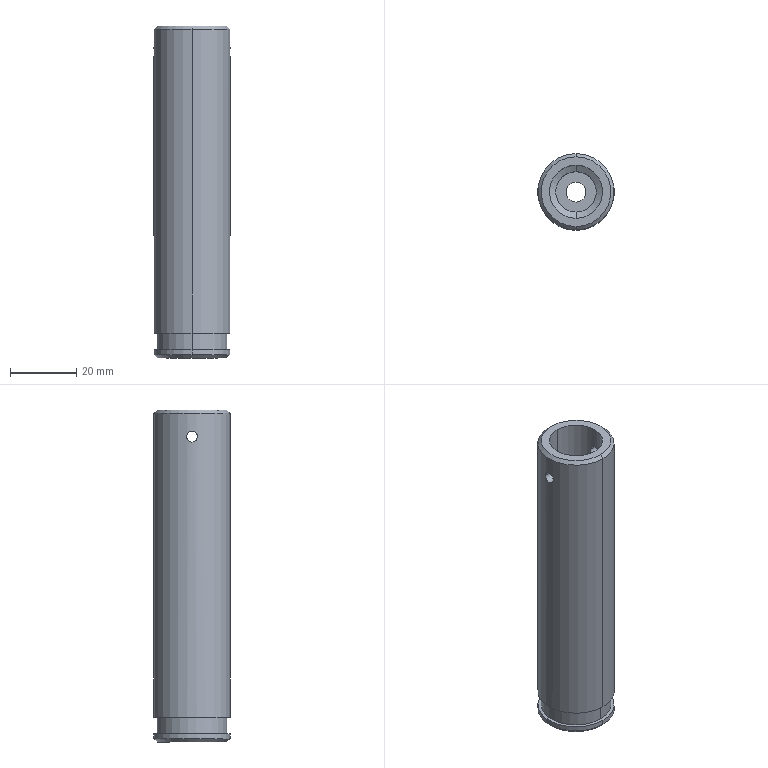Component | SolidWorks | DZ.KX.203-TC1505-20-18-05-98-1 | 1 solid | 30 faces | box 23 x 23 x 100 mm | volume 30575 mm3 | cylinder 18 | cone 6 | plane 6 | commonest cylinder face diameters 3.3 x4 23 x4 10.5 x2 21 x2 16 x2 12.2 x2 6 x2 | material Cast Stainless Steel
STEP:
#1=COLOUR_RGB('',0.7922,0.8196,0.9333);
#2=FILL_AREA_STYLE_COLOUR('',#1);
#3=FILL_AREA_STYLE('',(#2));
#4=SURFACE_STYLE_FILL_AREA(#3);
#5=SURFACE_SIDE_STYLE('',(#4));
#6=SURFACE_STYLE_USAGE(.BOTH.,#5);
#7=PRESENTATION_STYLE_ASSIGNMENT((#6));
#8=CARTESIAN_POINT('',(11.634,-31.784,4.53));
#9=VERTEX_POINT('',#8);
#10=CARTESIAN_POINT('',(11.634,-32.611,4.53));
#11=VERTEX_POINT('',#10);
#12=CARTESIAN_POINT('',(11.634,-32.197,4.53));
#13=DIRECTION('',(-0.,0.,1.));
#14=DIRECTION('',(0.,-1.,0.));
#15=AXIS2_PLACEMENT_3D('',#12,#13,#14);
#16=CIRCLE('',#15,0.4134);
#17=EDGE_CURVE('',#9,#11,#16,.T.);
#18=ORIENTED_EDGE('',*,*,#17,.F.);
#19=CARTESIAN_POINT('',(11.634,-31.744,4.491));
#20=VERTEX_POINT('',#19);
#21=CARTESIAN_POINT('',(11.634,-31.744,4.491));
#22=DIRECTION('',(-0.,0.7071,-0.7071));
#23=VECTOR('',#22,39.37);
#24=LINE('',#21,#23);
#25=EDGE_CURVE('',#9,#20,#24,.T.);
#26=ORIENTED_EDGE('',*,*,#25,.T.);
#27=CARTESIAN_POINT('',(11.634,-32.65,4.491));
#28=VERTEX_POINT('',#27);
#29=CARTESIAN_POINT('',(11.634,-32.197,4.491));
#30=DIRECTION('',(0.,-0.,-1.));
#31=DIRECTION('',(0.,-1.,0.));
#32=AXIS2_PLACEMENT_3D('',#29,#30,#31);
#33=CIRCLE('',#32,0.4528);
#34=EDGE_CURVE('',#28,#20,#33,.T.);
#35=ORIENTED_EDGE('',*,*,#34,.F.);
#36=CARTESIAN_POINT('',(11.634,-32.65,4.491));
#37=DIRECTION('',(0.,-0.7071,-0.7071));
#38=VECTOR('',#37,39.37);
#39=LINE('',#36,#38);
#40=EDGE_CURVE('',#11,#28,#39,.T.);
#41=ORIENTED_EDGE('',*,*,#40,.F.);
#42=EDGE_LOOP('',(#18,#26,#35,#41));
#43=FACE_OUTER_BOUND('',#42,.T.);
#44=CARTESIAN_POINT('',(11.634,-32.197,4.491));
#45=DIRECTION('',(0.,-0.,-1.));
#46=DIRECTION('',(0.,-1.,0.));
#47=AXIS2_PLACEMENT_3D('',#44,#45,#46);
#48=CONICAL_SURFACE('',#47,0.4528,0.7854);
#49=ADVANCED_FACE('',(#43),#48,.T.);
#50=CARTESIAN_POINT('',(11.634,-32.611,0.5929));
#51=VERTEX_POINT('',#50);
#52=CARTESIAN_POINT('',(11.634,-31.784,0.5929));
#53=VERTEX_POINT('',#52);
#54=CARTESIAN_POINT('',(11.634,-32.197,0.5929));
#55=DIRECTION('',(0.,-0.,-1.));
#56=DIRECTION('',(0.,-1.,0.));
#57=AXIS2_PLACEMENT_3D('',#54,#55,#56);
#58=CIRCLE('',#57,0.4134);
#59=EDGE_CURVE('',#51,#53,#58,.T.);
#60=ORIENTED_EDGE('',*,*,#59,.F.);
#61=CARTESIAN_POINT('',(11.634,-32.65,0.6323));
#62=VERTEX_POINT('',#61);
#63=CARTESIAN_POINT('',(11.634,-32.611,0.5929));
#64=DIRECTION('',(0.,-0.7071,0.7071));
#65=VECTOR('',#64,39.37);
#66=LINE('',#63,#65);
#67=EDGE_CURVE('',#51,#62,#66,.T.);
#68=ORIENTED_EDGE('',*,*,#67,.T.);
#69=CARTESIAN_POINT('',(11.634,-31.744,0.6323));
#70=VERTEX_POINT('',#69);
#71=CARTESIAN_POINT('',(11.634,-32.197,0.6323));
#72=DIRECTION('',(-0.,0.,1.));
#73=DIRECTION('',(0.,-1.,0.));
#74=AXIS2_PLACEMENT_3D('',#71,#72,#73);
#75=CIRCLE('',#74,0.4528);
#76=EDGE_CURVE('',#70,#62,#75,.T.);
#77=ORIENTED_EDGE('',*,*,#76,.F.);
#78=CARTESIAN_POINT('',(11.634,-31.784,0.5929));
#79=DIRECTION('',(-0.,0.7071,0.7071));
#80=VECTOR('',#79,39.37);
#81=LINE('',#78,#80);
#82=EDGE_CURVE('',#53,#70,#81,.T.);
#83=ORIENTED_EDGE('',*,*,#82,.F.);
#84=EDGE_LOOP('',(#60,#68,#77,#83));
#85=FACE_OUTER_BOUND('',#84,.T.);
#86=CARTESIAN_POINT('',(11.634,-32.197,0.5929));
#87=DIRECTION('',(-0.,0.,1.));
#88=DIRECTION('',(0.,1.,-0.));
#89=AXIS2_PLACEMENT_3D('',#86,#87,#88);
#90=CONICAL_SURFACE('',#89,0.4134,0.7854);
#91=ADVANCED_FACE('',(#85),#90,.T.);
#92=CARTESIAN_POINT('',(11.634,-31.99,1.183));
#93=VERTEX_POINT('',#92);
#94=CARTESIAN_POINT('',(11.634,-32.404,1.183));
#95=VERTEX_POINT('',#94);
#96=CARTESIAN_POINT('',(11.634,-32.197,1.183));
#97=DIRECTION('',(0.,-0.,-1.));
#98=DIRECTION('',(0.,-1.,0.));
#99=AXIS2_PLACEMENT_3D('',#96,#97,#98);
#100=CIRCLE('',#99,0.2067);
#101=EDGE_CURVE('',#93,#95,#100,.T.);
#102=ORIENTED_EDGE('',*,*,#101,.F.);
#103=CARTESIAN_POINT('',(11.634,-31.99,0.5929));
#104=VERTEX_POINT('',#103);
#105=CARTESIAN_POINT('',(11.634,-31.99,0.5929));
#106=DIRECTION('',(0.,-0.,-1.));
#107=VECTOR('',#106,39.37);
#108=LINE('',#105,#107);
#109=EDGE_CURVE('',#93,#104,#108,.T.);
#110=ORIENTED_EDGE('',*,*,#109,.T.);
#111=CARTESIAN_POINT('',(11.634,-32.404,0.5929));
#112=VERTEX_POINT('',#111);
#113=CARTESIAN_POINT('',(11.634,-32.197,0.5929));
#114=DIRECTION('',(0.,-0.,-1.));
#115=DIRECTION('',(0.,-1.,0.));
#116=AXIS2_PLACEMENT_3D('',#113,#114,#115);
#117=CIRCLE('',#116,0.2067);
#118=EDGE_CURVE('',#104,#112,#117,.T.);
#119=ORIENTED_EDGE('',*,*,#118,.T.);
#120=CARTESIAN_POINT('',(11.634,-32.404,0.5929));
#121=DIRECTION('',(0.,-0.,-1.));
#122=VECTOR('',#121,39.37);
#123=LINE('',#120,#122);
#124=EDGE_CURVE('',#95,#112,#123,.T.);
#125=ORIENTED_EDGE('',*,*,#124,.F.);
#126=EDGE_LOOP('',(#102,#110,#119,#125));
#127=FACE_OUTER_BOUND('',#126,.T.);
#128=CARTESIAN_POINT('',(11.634,-32.197,0.5929));
#129=DIRECTION('',(0.,-0.,-1.));
#130=DIRECTION('',(0.,-1.,0.));
#131=AXIS2_PLACEMENT_3D('',#128,#129,#130);
#132=CYLINDRICAL_SURFACE('',#131,0.2067);
#133=ADVANCED_FACE('',(#127),#132,.F.);
#134=CARTESIAN_POINT('',(11.634,-32.611,0.8882));
#135=VERTEX_POINT('',#134);
#136=CARTESIAN_POINT('',(11.634,-31.784,0.8882));
#137=VERTEX_POINT('',#136);
#138=CARTESIAN_POINT('',(11.634,-32.197,0.8882));
#139=DIRECTION('',(0.,-0.,-1.));
#140=DIRECTION('',(0.,-1.,0.));
#141=AXIS2_PLACEMENT_3D('',#138,#139,#140);
#142=CIRCLE('',#141,0.4134);
#143=EDGE_CURVE('',#135,#137,#142,.T.);
#144=ORIENTED_EDGE('',*,*,#143,.T.);
#145=CARTESIAN_POINT('',(11.634,-31.784,0.6913));
#146=VERTEX_POINT('',#145);
#147=CARTESIAN_POINT('',(11.634,-31.784,0.8882));
#148=DIRECTION('',(0.,-0.,-1.));
#149=VECTOR('',#148,39.37);
#150=LINE('',#147,#149);
#151=EDGE_CURVE('',#137,#146,#150,.T.);
#152=ORIENTED_EDGE('',*,*,#151,.T.);
#153=CARTESIAN_POINT('',(11.634,-32.611,0.6913));
#154=VERTEX_POINT('',#153);
#155=CARTESIAN_POINT('',(11.634,-32.197,0.6913));
#156=DIRECTION('',(0.,-0.,-1.));
#157=DIRECTION('',(0.,-1.,0.));
#158=AXIS2_PLACEMENT_3D('',#155,#156,#157);
#159=CIRCLE('',#158,0.4134);
#160=EDGE_CURVE('',#154,#146,#159,.T.);
#161=ORIENTED_EDGE('',*,*,#160,.F.);
#162=CARTESIAN_POINT('',(11.634,-32.611,0.8882));
#163=DIRECTION('',(0.,-0.,-1.));
#164=VECTOR('',#163,39.37);
#165=LINE('',#162,#164);
#166=EDGE_CURVE('',#135,#154,#165,.T.);
#167=ORIENTED_EDGE('',*,*,#166,.F.);
#168=EDGE_LOOP('',(#144,#152,#161,#167));
#169=FACE_OUTER_BOUND('',#168,.T.);
#170=CARTESIAN_POINT('',(11.634,-32.197,0.8882));
#171=DIRECTION('',(0.,-0.,-1.));
#172=DIRECTION('',(0.,-1.,0.));
#173=AXIS2_PLACEMENT_3D('',#170,#171,#172);
#174=CYLINDRICAL_SURFACE('',#173,0.4134);
#175=ADVANCED_FACE('',(#169),#174,.T.);
#176=CARTESIAN_POINT('',(12.082,-32.262,4.215));
#177=VERTEX_POINT('',#176);
#178=CARTESIAN_POINT('',(12.082,-32.132,4.215));
#179=VERTEX_POINT('',#178);
#180=CARTESIAN_POINT('',(12.082,-32.262,4.215));
#181=CARTESIAN_POINT('',(12.082,-32.262,4.219));
#182=CARTESIAN_POINT('',(12.082,-32.262,4.223));
#183=CARTESIAN_POINT('',(12.082,-32.26,4.232));
#184=CARTESIAN_POINT('',(12.082,-32.259,4.236));
#185=CARTESIAN_POINT('',(12.083,-32.255,4.244));
#186=CARTESIAN_POINT('',(12.083,-32.254,4.247));
#187=CARTESIAN_POINT('',(12.084,-32.249,4.255));
#188=CARTESIAN_POINT('',(12.084,-32.246,4.258));
#189=CARTESIAN_POINT('',(12.085,-32.237,4.267));
#190=CARTESIAN_POINT('',(12.085,-32.23,4.272));
#191=CARTESIAN_POINT('',(12.086,-32.214,4.278));
#192=CARTESIAN_POINT('',(12.087,-32.206,4.28));
#193=CARTESIAN_POINT('',(12.087,-32.193,4.28));
#194=CARTESIAN_POINT('',(12.087,-32.189,4.279));
#195=CARTESIAN_POINT('',(12.086,-32.18,4.278));
#196=CARTESIAN_POINT('',(12.086,-32.176,4.277));
#197=CARTESIAN_POINT('',(12.086,-32.168,4.273));
#198=CARTESIAN_POINT('',(12.085,-32.165,4.271));
#199=CARTESIAN_POINT('',(12.085,-32.157,4.267));
#200=CARTESIAN_POINT('',(12.085,-32.154,4.264));
#201=CARTESIAN_POINT('',(12.084,-32.145,4.255));
#202=CARTESIAN_POINT('',(12.083,-32.14,4.248));
#203=CARTESIAN_POINT('',(12.082,-32.134,4.232));
#204=CARTESIAN_POINT('',(12.082,-32.132,4.223));
#205=CARTESIAN_POINT('',(12.082,-32.132,4.215));
#206=B_SPLINE_CURVE_WITH_KNOTS('',3,(#180,#181,#182,#183,#184,#185,#186,#187,#188,#189,#190,#191,#192,#193,#194,#195,#196,#197,#198,#199,#200,#201,#202,#203,#204,#205),.UNSPECIFIED.,.F.,.F.,(4,2,2,2,2,2,2,2,2,2,2,2,4),(0.007748,0.008071,0.008394,0.008717,0.009039,0.009685,0.01033,0.01065,0.01098,0.0113,0.01162,0.01227,0.01291),.UNSPECIFIED.);
#207=EDGE_CURVE('',#177,#179,#206,.T.);
#208=ORIENTED_EDGE('',*,*,#207,.F.);
#209=CARTESIAN_POINT('',(11.942,-32.262,4.215));
#210=VERTEX_POINT('',#209);
#211=CARTESIAN_POINT('',(11.142,-32.262,4.215));
#212=DIRECTION('',(-1.,-0.,-0.));
#213=VECTOR('',#212,39.37);
#214=LINE('',#211,#213);
#215=EDGE_CURVE('',#177,#210,#214,.T.);
#216=ORIENTED_EDGE('',*,*,#215,.T.);
#217=CARTESIAN_POINT('',(11.942,-32.132,4.215));
#218=VERTEX_POINT('',#217);
#219=CARTESIAN_POINT('',(11.942,-32.132,4.215));
#220=CARTESIAN_POINT('',(11.942,-32.132,4.219));
#221=CARTESIAN_POINT('',(11.942,-32.133,4.223));
#222=CARTESIAN_POINT('',(11.942,-32.134,4.232));
#223=CARTESIAN_POINT('',(11.943,-32.135,4.236));
#224=CARTESIAN_POINT('',(11.943,-32.139,4.244));
#225=CARTESIAN_POINT('',(11.944,-32.141,4.248));
#226=CARTESIAN_POINT('',(11.945,-32.145,4.255));
#227=CARTESIAN_POINT('',(11.945,-32.148,4.258));
#228=CARTESIAN_POINT('',(11.946,-32.157,4.267));
#229=CARTESIAN_POINT('',(11.947,-32.164,4.272));
#230=CARTESIAN_POINT('',(11.948,-32.18,4.278));
#231=CARTESIAN_POINT('',(11.949,-32.189,4.28));
#232=CARTESIAN_POINT('',(11.949,-32.201,4.28));
#233=CARTESIAN_POINT('',(11.949,-32.206,4.279));
#234=CARTESIAN_POINT('',(11.948,-32.214,4.278));
#235=CARTESIAN_POINT('',(11.948,-32.218,4.277));
#236=CARTESIAN_POINT('',(11.947,-32.23,4.272));
#237=CARTESIAN_POINT('',(11.946,-32.237,4.267));
#238=CARTESIAN_POINT('',(11.945,-32.246,4.258));
#239=CARTESIAN_POINT('',(11.945,-32.249,4.255));
#240=CARTESIAN_POINT('',(11.944,-32.253,4.248));
#241=CARTESIAN_POINT('',(11.943,-32.255,4.244));
#242=CARTESIAN_POINT('',(11.943,-32.259,4.236));
#243=CARTESIAN_POINT('',(11.942,-32.26,4.232));
#244=CARTESIAN_POINT('',(11.942,-32.262,4.224));
#245=CARTESIAN_POINT('',(11.942,-32.262,4.219));
#246=CARTESIAN_POINT('',(11.942,-32.262,4.215));
#247=B_SPLINE_CURVE_WITH_KNOTS('',3,(#219,#220,#221,#222,#223,#224,#225,#226,#227,#228,#229,#230,#231,#232,#233,#234,#235,#236,#237,#238,#239,#240,#241,#242,#243,#244,#245,#246),.UNSPECIFIED.,.F.,.F.,(4,2,2,2,2,2,2,2,2,2,2,2,2,4),(0.,0.0003233,0.0006466,0.0009699,0.001293,0.00194,0.002586,0.00291,0.003233,0.003879,0.004203,0.004526,0.004849,0.005173),.UNSPECIFIED.);
#248=EDGE_CURVE('',#218,#210,#247,.T.);
#249=ORIENTED_EDGE('',*,*,#248,.F.);
#250=CARTESIAN_POINT('',(11.142,-32.132,4.215));
#251=DIRECTION('',(-1.,-0.,-0.));
#252=VECTOR('',#251,39.37);
#253=LINE('',#250,#252);
#254=EDGE_CURVE('',#179,#218,#253,.T.);
#255=ORIENTED_EDGE('',*,*,#254,.F.);
#256=EDGE_LOOP('',(#208,#216,#249,#255));
#257=FACE_OUTER_BOUND('',#256,.T.);
#258=CARTESIAN_POINT('',(11.142,-32.197,4.215));
#259=DIRECTION('',(-1.,-0.,-0.));
#260=DIRECTION('',(0.,1.,0.));
#261=AXIS2_PLACEMENT_3D('',#258,#259,#260);
#262=CYLINDRICAL_SURFACE('',#261,0.06496);
#263=ADVANCED_FACE('',(#257),#262,.F.);
#264=CARTESIAN_POINT('',(11.326,-32.262,4.215));
#265=VERTEX_POINT('',#264);
#266=CARTESIAN_POINT('',(11.326,-32.132,4.215));
#267=VERTEX_POINT('',#266);
#268=CARTESIAN_POINT('',(11.326,-32.262,4.215));
#269=CARTESIAN_POINT('',(11.326,-32.262,4.223));
#270=CARTESIAN_POINT('',(11.325,-32.26,4.232));
#271=CARTESIAN_POINT('',(11.324,-32.256,4.244));
#272=CARTESIAN_POINT('',(11.324,-32.253,4.248));
#273=CARTESIAN_POINT('',(11.323,-32.249,4.255));
#274=CARTESIAN_POINT('',(11.323,-32.246,4.258));
#275=CARTESIAN_POINT('',(11.322,-32.24,4.264));
#276=CARTESIAN_POINT('',(11.321,-32.237,4.267));
#277=CARTESIAN_POINT('',(11.321,-32.23,4.271));
#278=CARTESIAN_POINT('',(11.32,-32.226,4.273));
#279=CARTESIAN_POINT('',(11.319,-32.214,4.278));
#280=CARTESIAN_POINT('',(11.319,-32.206,4.28));
#281=CARTESIAN_POINT('',(11.319,-32.193,4.28));
#282=CARTESIAN_POINT('',(11.319,-32.189,4.279));
#283=CARTESIAN_POINT('',(11.319,-32.18,4.278));
#284=CARTESIAN_POINT('',(11.32,-32.176,4.277));
#285=CARTESIAN_POINT('',(11.32,-32.168,4.273));
#286=CARTESIAN_POINT('',(11.321,-32.165,4.271));
#287=CARTESIAN_POINT('',(11.321,-32.158,4.267));
#288=CARTESIAN_POINT('',(11.322,-32.154,4.264));
#289=CARTESIAN_POINT('',(11.323,-32.145,4.255));
#290=CARTESIAN_POINT('',(11.324,-32.14,4.248));
#291=CARTESIAN_POINT('',(11.325,-32.136,4.236));
#292=CARTESIAN_POINT('',(11.325,-32.134,4.232));
#293=CARTESIAN_POINT('',(11.326,-32.133,4.223));
#294=CARTESIAN_POINT('',(11.326,-32.132,4.219));
#295=CARTESIAN_POINT('',(11.326,-32.132,4.215));
#296=B_SPLINE_CURVE_WITH_KNOTS('',3,(#268,#269,#270,#271,#272,#273,#274,#275,#276,#277,#278,#279,#280,#281,#282,#283,#284,#285,#286,#287,#288,#289,#290,#291,#292,#293,#294,#295),.UNSPECIFIED.,.F.,.F.,(4,2,2,2,2,2,2,2,2,2,2,2,2,4),(0.005173,0.005819,0.006142,0.006465,0.006789,0.007112,0.007758,0.008081,0.008405,0.008728,0.009051,0.009697,0.01002,0.01034),.UNSPECIFIED.);
#297=EDGE_CURVE('',#265,#267,#296,.T.);
#298=ORIENTED_EDGE('',*,*,#297,.F.);
#299=CARTESIAN_POINT('',(11.186,-32.262,4.215));
#300=VERTEX_POINT('',#299);
#301=CARTESIAN_POINT('',(11.142,-32.262,4.215));
#302=DIRECTION('',(-1.,-0.,-0.));
#303=VECTOR('',#302,39.37);
#304=LINE('',#301,#303);
#305=EDGE_CURVE('',#265,#300,#304,.T.);
#306=ORIENTED_EDGE('',*,*,#305,.T.);
#307=CARTESIAN_POINT('',(11.186,-32.132,4.215));
#308=VERTEX_POINT('',#307);
#309=CARTESIAN_POINT('',(11.186,-32.132,4.215));
#310=CARTESIAN_POINT('',(11.186,-32.132,4.219));
#311=CARTESIAN_POINT('',(11.186,-32.133,4.223));
#312=CARTESIAN_POINT('',(11.185,-32.134,4.232));
#313=CARTESIAN_POINT('',(11.185,-32.135,4.236));
#314=CARTESIAN_POINT('',(11.185,-32.139,4.244));
#315=CARTESIAN_POINT('',(11.185,-32.141,4.247));
#316=CARTESIAN_POINT('',(11.184,-32.145,4.255));
#317=CARTESIAN_POINT('',(11.184,-32.148,4.258));
#318=CARTESIAN_POINT('',(11.183,-32.157,4.267));
#319=CARTESIAN_POINT('',(11.182,-32.164,4.272));
#320=CARTESIAN_POINT('',(11.181,-32.18,4.278));
#321=CARTESIAN_POINT('',(11.181,-32.189,4.28));
#322=CARTESIAN_POINT('',(11.181,-32.201,4.28));
#323=CARTESIAN_POINT('',(11.181,-32.206,4.279));
#324=CARTESIAN_POINT('',(11.181,-32.214,4.278));
#325=CARTESIAN_POINT('',(11.182,-32.218,4.277));
#326=CARTESIAN_POINT('',(11.182,-32.226,4.273));
#327=CARTESIAN_POINT('',(11.182,-32.23,4.271));
#328=CARTESIAN_POINT('',(11.183,-32.237,4.267));
#329=CARTESIAN_POINT('',(11.183,-32.24,4.264));
#330=CARTESIAN_POINT('',(11.184,-32.246,4.258));
#331=CARTESIAN_POINT('',(11.184,-32.249,4.255));
#332=CARTESIAN_POINT('',(11.185,-32.253,4.248));
#333=CARTESIAN_POINT('',(11.185,-32.256,4.244));
#334=CARTESIAN_POINT('',(11.185,-32.259,4.236));
#335=CARTESIAN_POINT('',(11.185,-32.26,4.232));
#336=CARTESIAN_POINT('',(11.186,-32.262,4.223));
#337=CARTESIAN_POINT('',(11.186,-32.262,4.219));
#338=CARTESIAN_POINT('',(11.186,-32.262,4.215));
#339=B_SPLINE_CURVE_WITH_KNOTS('',3,(#309,#310,#311,#312,#313,#314,#315,#316,#317,#318,#319,#320,#321,#322,#323,#324,#325,#326,#327,#328,#329,#330,#331,#332,#333,#334,#335,#336,#337,#338),.UNSPECIFIED.,.F.,.F.,(4,2,2,2,2,2,2,2,2,2,2,2,2,2,4),(0.,0.0003228,0.0006457,0.0009685,0.001291,0.001937,0.002583,0.002905,0.003228,0.003551,0.003874,0.004197,0.00452,0.004842,0.005165),.UNSPECIFIED.);
#340=EDGE_CURVE('',#308,#300,#339,.T.);
#341=ORIENTED_EDGE('',*,*,#340,.F.);
#342=CARTESIAN_POINT('',(11.142,-32.132,4.215));
#343=DIRECTION('',(-1.,-0.,-0.));
#344=VECTOR('',#343,39.37);
#345=LINE('',#342,#344);
#346=EDGE_CURVE('',#267,#308,#345,.T.);
#347=ORIENTED_EDGE('',*,*,#346,.F.);
#348=EDGE_LOOP('',(#298,#306,#341,#347));
#349=FACE_OUTER_BOUND('',#348,.T.);
#350=CARTESIAN_POINT('',(11.142,-32.197,4.215));
#351=DIRECTION('',(-1.,-0.,-0.));
#352=DIRECTION('',(0.,1.,0.));
#353=AXIS2_PLACEMENT_3D('',#350,#351,#352);
#354=CYLINDRICAL_SURFACE('',#353,0.06496);
#355=ADVANCED_FACE('',(#349),#354,.F.);
#356=ORIENTED_EDGE('',*,*,#248,.T.);
#357=CARTESIAN_POINT('',(11.942,-32.262,4.215));
#358=CARTESIAN_POINT('',(11.942,-32.262,4.206));
#359=CARTESIAN_POINT('',(11.942,-32.26,4.198));
#360=CARTESIAN_POINT('',(11.943,-32.256,4.186));
#361=CARTESIAN_POINT('',(11.944,-32.253,4.182));
#362=CARTESIAN_POINT('',(11.945,-32.249,4.175));
#363=CARTESIAN_POINT('',(11.945,-32.246,4.172));
#364=CARTESIAN_POINT('',(11.946,-32.24,4.166));
#365=CARTESIAN_POINT('',(11.946,-32.237,4.163));
#366=CARTESIAN_POINT('',(11.947,-32.23,4.159));
#367=CARTESIAN_POINT('',(11.948,-32.226,4.157));
#368=CARTESIAN_POINT('',(11.948,-32.214,4.152));
#369=CARTESIAN_POINT('',(11.949,-32.206,4.15));
#370=CARTESIAN_POINT('',(11.949,-32.193,4.15));
#371=CARTESIAN_POINT('',(11.949,-32.189,4.15));
#372=CARTESIAN_POINT('',(11.948,-32.18,4.152));
#373=CARTESIAN_POINT('',(11.948,-32.176,4.153));
#374=CARTESIAN_POINT('',(11.948,-32.168,4.157));
#375=CARTESIAN_POINT('',(11.947,-32.165,4.159));
#376=CARTESIAN_POINT('',(11.946,-32.158,4.163));
#377=CARTESIAN_POINT('',(11.946,-32.154,4.166));
#378=CARTESIAN_POINT('',(11.945,-32.145,4.175));
#379=CARTESIAN_POINT('',(11.944,-32.14,4.182));
#380=CARTESIAN_POINT('',(11.943,-32.136,4.194));
#381=CARTESIAN_POINT('',(11.942,-32.134,4.198));
#382=CARTESIAN_POINT('',(11.942,-32.133,4.206));
#383=CARTESIAN_POINT('',(11.942,-32.132,4.211));
#384=CARTESIAN_POINT('',(11.942,-32.132,4.215));
#385=B_SPLINE_CURVE_WITH_KNOTS('',3,(#357,#358,#359,#360,#361,#362,#363,#364,#365,#366,#367,#368,#369,#370,#371,#372,#373,#374,#375,#376,#377,#378,#379,#380,#381,#382,#383,#384),.UNSPECIFIED.,.F.,.F.,(4,2,2,2,2,2,2,2,2,2,2,2,2,4),(0.005173,0.005819,0.006142,0.006465,0.006789,0.007112,0.007758,0.008081,0.008405,0.008728,0.009051,0.009697,0.01002,0.01034),.UNSPECIFIED.);
#386=EDGE_CURVE('',#210,#218,#385,.T.);
#387=ORIENTED_EDGE('',*,*,#386,.T.);
#388=EDGE_LOOP('',(#356,#387));
#389=FACE_BOUND('',#388,.T.);
#390=CARTESIAN_POINT('',(11.634,-32.512,3.861));
#391=VERTEX_POINT('',#390);
#392=CARTESIAN_POINT('',(11.634,-31.882,3.861));
#393=VERTEX_POINT('',#392);
#394=CARTESIAN_POINT('',(11.634,-32.197,3.861));
#395=DIRECTION('',(-0.,0.,1.));
#396=DIRECTION('',(0.,1.,-0.));
#397=AXIS2_PLACEMENT_3D('',#394,#395,#396);
#398=CIRCLE('',#397,0.315);
#399=EDGE_CURVE('',#391,#393,#398,.T.);
#400=ORIENTED_EDGE('',*,*,#399,.F.);
#401=CARTESIAN_POINT('',(11.634,-32.512,4.53));
#402=VERTEX_POINT('',#401);
#403=CARTESIAN_POINT('',(11.634,-32.512,4.53));
#404=DIRECTION('',(-0.,0.,1.));
#405=VECTOR('',#404,39.37);
#406=LINE('',#403,#405);
#407=EDGE_CURVE('',#391,#402,#406,.T.);
#408=ORIENTED_EDGE('',*,*,#407,.T.);
#409=CARTESIAN_POINT('',(11.634,-31.882,4.53));
#410=VERTEX_POINT('',#409);
#411=CARTESIAN_POINT('',(11.634,-32.197,4.53));
#412=DIRECTION('',(-0.,0.,1.));
#413=DIRECTION('',(0.,1.,-0.));
#414=AXIS2_PLACEMENT_3D('',#411,#412,#413);
#415=CIRCLE('',#414,0.315);
#416=EDGE_CURVE('',#402,#410,#415,.T.);
#417=ORIENTED_EDGE('',*,*,#416,.T.);
#418=CARTESIAN_POINT('',(11.634,-31.882,4.53));
#419=DIRECTION('',(-0.,0.,1.));
#420=VECTOR('',#419,39.37);
#421=LINE('',#418,#420);
#422=EDGE_CURVE('',#393,#410,#421,.T.);
#423=ORIENTED_EDGE('',*,*,#422,.F.);
#424=EDGE_LOOP('',(#400,#408,#417,#423));
#425=FACE_OUTER_BOUND('',#424,.T.);
#426=CARTESIAN_POINT('',(11.634,-32.197,4.53));
#427=DIRECTION('',(-0.,0.,1.));
#428=DIRECTION('',(0.,1.,-0.));
#429=AXIS2_PLACEMENT_3D('',#426,#427,#428);
#430=CYLINDRICAL_SURFACE('',#429,0.315);
#431=ADVANCED_FACE('',(#389,#425),#430,.F.);
#432=CARTESIAN_POINT('',(11.634,-32.437,3.816));
#433=VERTEX_POINT('',#432);
#434=CARTESIAN_POINT('',(11.634,-31.957,3.816));
#435=VERTEX_POINT('',#434);
#436=CARTESIAN_POINT('',(11.634,-32.197,3.816));
#437=DIRECTION('',(-0.,0.,1.));
#438=DIRECTION('',(0.,1.,-0.));
#439=AXIS2_PLACEMENT_3D('',#436,#437,#438);
#440=CIRCLE('',#439,0.2402);
#441=EDGE_CURVE('',#433,#435,#440,.T.);
#442=ORIENTED_EDGE('',*,*,#441,.F.);
#443=CARTESIAN_POINT('',(11.634,-32.512,3.861));
#444=DIRECTION('',(0.,-0.8572,0.515));
#445=VECTOR('',#444,39.37);
#446=LINE('',#443,#445);
#447=EDGE_CURVE('',#433,#391,#446,.T.);
#448=ORIENTED_EDGE('',*,*,#447,.T.);
#449=ORIENTED_EDGE('',*,*,#399,.T.);
#450=CARTESIAN_POINT('',(11.634,-31.882,3.861));
#451=DIRECTION('',(-0.,0.8572,0.515));
#452=VECTOR('',#451,39.37);
#453=LINE('',#450,#452);
#454=EDGE_CURVE('',#435,#393,#453,.T.);
#455=ORIENTED_EDGE('',*,*,#454,.F.);
#456=EDGE_LOOP('',(#442,#448,#449,#455));
#457=FACE_OUTER_BOUND('',#456,.T.);
#458=CARTESIAN_POINT('',(11.634,-32.197,3.861));
#459=DIRECTION('',(-0.,0.,1.));
#460=DIRECTION('',(0.,1.,-0.));
#461=AXIS2_PLACEMENT_3D('',#458,#459,#460);
#462=CONICAL_SURFACE('',#461,0.315,1.03);
#463=ADVANCED_FACE('',(#457),#462,.F.);
#464=CARTESIAN_POINT('',(11.634,-32.437,2.168));
#465=VERTEX_POINT('',#464);
#466=CARTESIAN_POINT('',(11.634,-31.957,2.168));
#467=VERTEX_POINT('',#466);
#468=CARTESIAN_POINT('',(11.634,-32.197,2.168));
#469=DIRECTION('',(-0.,0.,1.));
#470=DIRECTION('',(0.,1.,-0.));
#471=AXIS2_PLACEMENT_3D('',#468,#469,#470);
#472=CIRCLE('',#471,0.2402);
#473=EDGE_CURVE('',#465,#467,#472,.T.);
#474=ORIENTED_EDGE('',*,*,#473,.F.);
#475=CARTESIAN_POINT('',(11.634,-32.437,4.53));
#476=DIRECTION('',(-0.,0.,1.));
#477=VECTOR('',#476,39.37);
#478=LINE('',#475,#477);
#479=EDGE_CURVE('',#465,#433,#478,.T.);
#480=ORIENTED_EDGE('',*,*,#479,.T.);
#481=ORIENTED_EDGE('',*,*,#441,.T.);
#482=CARTESIAN_POINT('',(11.634,-31.957,4.53));
#483=DIRECTION('',(-0.,0.,1.));
#484=VECTOR('',#483,39.37);
#485=LINE('',#482,#484);
#486=EDGE_CURVE('',#467,#435,#485,.T.);
#487=ORIENTED_EDGE('',*,*,#486,.F.);
#488=EDGE_LOOP('',(#474,#480,#481,#487));
#489=FACE_OUTER_BOUND('',#488,.T.);
#490=CARTESIAN_POINT('',(11.634,-32.197,4.53));
#491=DIRECTION('',(-0.,0.,1.));
#492=DIRECTION('',(0.,1.,-0.));
#493=AXIS2_PLACEMENT_3D('',#490,#491,#492);
#494=CYLINDRICAL_SURFACE('',#493,0.2402);
#495=ADVANCED_FACE('',(#489),#494,.F.);
#496=CARTESIAN_POINT('',(11.634,-32.079,1.183));
#497=VERTEX_POINT('',#496);
#498=CARTESIAN_POINT('',(11.634,-32.315,1.183));
#499=VERTEX_POINT('',#498);
#500=CARTESIAN_POINT('',(11.634,-32.197,1.183));
#501=DIRECTION('',(0.,-0.,-1.));
#502=DIRECTION('',(0.,1.,-0.));
#503=AXIS2_PLACEMENT_3D('',#500,#501,#502);
#504=CIRCLE('',#503,0.1181);
#505=EDGE_CURVE('',#497,#499,#504,.T.);
#506=ORIENTED_EDGE('',*,*,#505,.T.);
#507=CARTESIAN_POINT('',(11.634,-32.315,2.168));
#508=VERTEX_POINT('',#507);
#509=CARTESIAN_POINT('',(11.634,-32.315,4.53));
#510=DIRECTION('',(-0.,0.,1.));
#511=VECTOR('',#510,39.37);
#512=LINE('',#509,#511);
#513=EDGE_CURVE('',#499,#508,#512,.T.);
#514=ORIENTED_EDGE('',*,*,#513,.T.);
#515=CARTESIAN_POINT('',(11.634,-32.079,2.168));
#516=VERTEX_POINT('',#515);
#517=CARTESIAN_POINT('',(11.634,-32.197,2.168));
#518=DIRECTION('',(-0.,0.,1.));
#519=DIRECTION('',(0.,1.,-0.));
#520=AXIS2_PLACEMENT_3D('',#517,#518,#519);
#521=CIRCLE('',#520,0.1181);
#522=EDGE_CURVE('',#508,#516,#521,.T.);
#523=ORIENTED_EDGE('',*,*,#522,.T.);
#524=CARTESIAN_POINT('',(11.634,-32.079,4.53));
#525=DIRECTION('',(-0.,0.,1.));
#526=VECTOR('',#525,39.37);
#527=LINE('',#524,#526);
#528=EDGE_CURVE('',#497,#516,#527,.T.);
#529=ORIENTED_EDGE('',*,*,#528,.F.);
#530=EDGE_LOOP('',(#506,#514,#523,#529));
#531=FACE_OUTER_BOUND('',#530,.T.);
#532=CARTESIAN_POINT('',(11.634,-32.197,4.53));
#533=DIRECTION('',(-0.,0.,1.));
#534=DIRECTION('',(0.,1.,-0.));
#535=AXIS2_PLACEMENT_3D('',#532,#533,#534);
#536=CYLINDRICAL_SURFACE('',#535,0.1181);
#537=ADVANCED_FACE('',(#531),#536,.F.);
#538=ORIENTED_EDGE('',*,*,#76,.T.);
#539=CARTESIAN_POINT('',(11.634,-32.65,0.6913));
#540=VERTEX_POINT('',#539);
#541=CARTESIAN_POINT('',(11.634,-32.65,0.5929));
#542=DIRECTION('',(-0.,0.,1.));
#543=VECTOR('',#542,39.37);
#544=LINE('',#541,#543);
#545=EDGE_CURVE('',#62,#540,#544,.T.);
#546=ORIENTED_EDGE('',*,*,#545,.T.);
#547=CARTESIAN_POINT('',(11.634,-31.744,0.6913));
#548=VERTEX_POINT('',#547);
#549=CARTESIAN_POINT('',(11.634,-32.197,0.6913));
#550=DIRECTION('',(0.,-0.,-1.));
#551=DIRECTION('',(0.,-1.,0.));
#552=AXIS2_PLACEMENT_3D('',#549,#550,#551);
#553=CIRCLE('',#552,0.4528);
#554=EDGE_CURVE('',#540,#548,#553,.T.);
#555=ORIENTED_EDGE('',*,*,#554,.T.);
#556=CARTESIAN_POINT('',(11.634,-31.744,0.5929));
#557=DIRECTION('',(-0.,0.,1.));
#558=VECTOR('',#557,39.37);
#559=LINE('',#556,#558);
#560=EDGE_CURVE('',#70,#548,#559,.T.);
#561=ORIENTED_EDGE('',*,*,#560,.F.);
#562=EDGE_LOOP('',(#538,#546,#555,#561));
#563=FACE_OUTER_BOUND('',#562,.T.);
#564=CARTESIAN_POINT('',(11.634,-32.197,0.5929));
#565=DIRECTION('',(-0.,0.,1.));
#566=DIRECTION('',(-0.,1.,-0.));
#567=AXIS2_PLACEMENT_3D('',#564,#565,#566);
#568=CYLINDRICAL_SURFACE('',#567,0.4528);
#569=ADVANCED_FACE('',(#563),#568,.T.);
#570=ORIENTED_EDGE('',*,*,#340,.T.);
#571=CARTESIAN_POINT('',(11.186,-32.262,4.215));
#572=CARTESIAN_POINT('',(11.186,-32.262,4.206));
#573=CARTESIAN_POINT('',(11.186,-32.26,4.198));
#574=CARTESIAN_POINT('',(11.185,-32.254,4.182));
#575=CARTESIAN_POINT('',(11.184,-32.249,4.175));
#576=CARTESIAN_POINT('',(11.183,-32.24,4.166));
#577=CARTESIAN_POINT('',(11.183,-32.237,4.163));
#578=CARTESIAN_POINT('',(11.182,-32.23,4.159));
#579=CARTESIAN_POINT('',(11.182,-32.226,4.157));
#580=CARTESIAN_POINT('',(11.182,-32.218,4.153));
#581=CARTESIAN_POINT('',(11.181,-32.214,4.152));
#582=CARTESIAN_POINT('',(11.181,-32.206,4.15));
#583=CARTESIAN_POINT('',(11.181,-32.201,4.15));
#584=CARTESIAN_POINT('',(11.181,-32.193,4.15));
#585=CARTESIAN_POINT('',(11.181,-32.189,4.15));
#586=CARTESIAN_POINT('',(11.181,-32.18,4.152));
#587=CARTESIAN_POINT('',(11.182,-32.176,4.153));
#588=CARTESIAN_POINT('',(11.182,-32.168,4.157));
#589=CARTESIAN_POINT('',(11.182,-32.165,4.159));
#590=CARTESIAN_POINT('',(11.183,-32.158,4.163));
#591=CARTESIAN_POINT('',(11.183,-32.154,4.166));
#592=CARTESIAN_POINT('',(11.184,-32.145,4.175));
#593=CARTESIAN_POINT('',(11.185,-32.14,4.182));
#594=CARTESIAN_POINT('',(11.186,-32.134,4.198));
#595=CARTESIAN_POINT('',(11.186,-32.132,4.206));
#596=CARTESIAN_POINT('',(11.186,-32.132,4.215));
#597=B_SPLINE_CURVE_WITH_KNOTS('',3,(#571,#572,#573,#574,#575,#576,#577,#578,#579,#580,#581,#582,#583,#584,#585,#586,#587,#588,#589,#590,#591,#592,#593,#594,#595,#596),.UNSPECIFIED.,.F.,.F.,(4,2,2,2,2,2,2,2,2,2,2,2,4),(0.005165,0.005811,0.006456,0.006779,0.007102,0.007425,0.007747,0.00807,0.008393,0.008716,0.009038,0.009684,0.01033),.UNSPECIFIED.);
#598=EDGE_CURVE('',#300,#308,#597,.T.);
#599=ORIENTED_EDGE('',*,*,#598,.T.);
#600=EDGE_LOOP('',(#570,#599));
#601=FACE_BOUND('',#600,.T.);
#602=CARTESIAN_POINT('',(11.634,-32.65,0.8882));
#603=VERTEX_POINT('',#602);
#604=CARTESIAN_POINT('',(11.634,-31.744,0.8882));
#605=VERTEX_POINT('',#604);
#606=CARTESIAN_POINT('',(11.634,-32.197,0.8882));
#607=DIRECTION('',(0.,-0.,-1.));
#608=DIRECTION('',(0.,-1.,0.));
#609=AXIS2_PLACEMENT_3D('',#606,#607,#608);
#610=CIRCLE('',#609,0.4528);
#611=EDGE_CURVE('',#603,#605,#610,.T.);
#612=ORIENTED_EDGE('',*,*,#611,.F.);
#613=CARTESIAN_POINT('',(11.634,-32.65,0.5929));
#614=DIRECTION('',(-0.,0.,1.));
#615=VECTOR('',#614,39.37);
#616=LINE('',#613,#615);
#617=EDGE_CURVE('',#603,#28,#616,.T.);
#618=ORIENTED_EDGE('',*,*,#617,.T.);
#619=ORIENTED_EDGE('',*,*,#34,.T.);
#620=CARTESIAN_POINT('',(11.634,-31.744,0.5929));
#621=DIRECTION('',(-0.,0.,1.));
#622=VECTOR('',#621,39.37);
#623=LINE('',#620,#622);
#624=EDGE_CURVE('',#605,#20,#623,.T.);
#625=ORIENTED_EDGE('',*,*,#624,.F.);
#626=EDGE_LOOP('',(#612,#618,#619,#625));
#627=FACE_OUTER_BOUND('',#626,.T.);
#628=CARTESIAN_POINT('',(11.634,-32.197,0.5929));
#629=DIRECTION('',(-0.,0.,1.));
#630=DIRECTION('',(-0.,1.,-0.));
#631=AXIS2_PLACEMENT_3D('',#628,#629,#630);
#632=CYLINDRICAL_SURFACE('',#631,0.4528);
#633=ADVANCED_FACE('',(#601,#627),#632,.T.);
#634=ORIENTED_EDGE('',*,*,#617,.F.);
#635=CARTESIAN_POINT('',(11.634,-32.197,0.8882));
#636=DIRECTION('',(0.,-0.,-1.));
#637=DIRECTION('',(0.,-1.,0.));
#638=AXIS2_PLACEMENT_3D('',#635,#636,#637);
#639=CIRCLE('',#638,0.4528);
#640=EDGE_CURVE('',#605,#603,#639,.T.);
#641=ORIENTED_EDGE('',*,*,#640,.F.);
#642=ORIENTED_EDGE('',*,*,#624,.T.);
#643=CARTESIAN_POINT('',(11.634,-32.197,4.491));
#644=DIRECTION('',(0.,-0.,-1.));
#645=DIRECTION('',(0.,-1.,0.));
#646=AXIS2_PLACEMENT_3D('',#643,#644,#645);
#647=CIRCLE('',#646,0.4528);
#648=EDGE_CURVE('',#20,#28,#647,.T.);
#649=ORIENTED_EDGE('',*,*,#648,.T.);
#650=EDGE_LOOP('',(#634,#641,#642,#649));
#651=FACE_OUTER_BOUND('',#650,.T.);
#652=CARTESIAN_POINT('',(12.082,-32.132,4.215));
#653=CARTESIAN_POINT('',(12.082,-32.132,4.211));
#654=CARTESIAN_POINT('',(12.082,-32.133,4.206));
#655=CARTESIAN_POINT('',(12.082,-32.134,4.198));
#656=CARTESIAN_POINT('',(12.082,-32.135,4.194));
#657=CARTESIAN_POINT('',(12.083,-32.139,4.186));
#658=CARTESIAN_POINT('',(12.083,-32.141,4.182));
#659=CARTESIAN_POINT('',(12.084,-32.145,4.175));
#660=CARTESIAN_POINT('',(12.084,-32.148,4.172));
#661=CARTESIAN_POINT('',(12.085,-32.154,4.166));
#662=CARTESIAN_POINT('',(12.085,-32.158,4.163));
#663=CARTESIAN_POINT('',(12.085,-32.165,4.159));
#664=CARTESIAN_POINT('',(12.086,-32.168,4.157));
#665=CARTESIAN_POINT('',(12.086,-32.176,4.153));
#666=CARTESIAN_POINT('',(12.086,-32.18,4.152));
#667=CARTESIAN_POINT('',(12.087,-32.189,4.15));
#668=CARTESIAN_POINT('',(12.087,-32.193,4.15));
#669=CARTESIAN_POINT('',(12.087,-32.206,4.15));
#670=CARTESIAN_POINT('',(12.086,-32.214,4.152));
#671=CARTESIAN_POINT('',(12.085,-32.23,4.158));
#672=CARTESIAN_POINT('',(12.085,-32.237,4.163));
#673=CARTESIAN_POINT('',(12.084,-32.246,4.172));
#674=CARTESIAN_POINT('',(12.084,-32.249,4.175));
#675=CARTESIAN_POINT('',(12.083,-32.253,4.182));
#676=CARTESIAN_POINT('',(12.083,-32.255,4.186));
#677=CARTESIAN_POINT('',(12.082,-32.259,4.194));
#678=CARTESIAN_POINT('',(12.082,-32.26,4.198));
#679=CARTESIAN_POINT('',(12.082,-32.262,4.206));
#680=CARTESIAN_POINT('',(12.082,-32.262,4.211));
#681=CARTESIAN_POINT('',(12.082,-32.262,4.215));
#682=B_SPLINE_CURVE_WITH_KNOTS('',3,(#652,#653,#654,#655,#656,#657,#658,#659,#660,#661,#662,#663,#664,#665,#666,#667,#668,#669,#670,#671,#672,#673,#674,#675,#676,#677,#678,#679,#680,#681),.UNSPECIFIED.,.F.,.F.,(4,2,2,2,2,2,2,2,2,2,2,2,2,2,4),(0.002583,0.002906,0.003229,0.003552,0.003875,0.004197,0.00452,0.004843,0.005166,0.005812,0.006457,0.00678,0.007103,0.007426,0.007748),.UNSPECIFIED.);
#683=EDGE_CURVE('',#179,#177,#682,.T.);
#684=ORIENTED_EDGE('',*,*,#683,.T.);
#685=ORIENTED_EDGE('',*,*,#207,.T.);
#686=EDGE_LOOP('',(#684,#685));
#687=FACE_BOUND('',#686,.T.);
#688=CARTESIAN_POINT('',(11.634,-32.197,0.5929));
#689=DIRECTION('',(-0.,0.,1.));
#690=DIRECTION('',(-0.,1.,-0.));
#691=AXIS2_PLACEMENT_3D('',#688,#689,#690);
#692=CYLINDRICAL_SURFACE('',#691,0.4528);
#693=ADVANCED_FACE('',(#651,#687),#692,.T.);
#694=ORIENTED_EDGE('',*,*,#545,.F.);
#695=CARTESIAN_POINT('',(11.634,-32.197,0.6323));
#696=DIRECTION('',(-0.,0.,1.));
#697=DIRECTION('',(0.,-1.,0.));
#698=AXIS2_PLACEMENT_3D('',#695,#696,#697);
#699=CIRCLE('',#698,0.4528);
#700=EDGE_CURVE('',#62,#70,#699,.T.);
#701=ORIENTED_EDGE('',*,*,#700,.T.);
#702=ORIENTED_EDGE('',*,*,#560,.T.);
#703=CARTESIAN_POINT('',(11.634,-32.197,0.6913));
#704=DIRECTION('',(0.,-0.,-1.));
#705=DIRECTION('',(0.,-1.,0.));
#706=AXIS2_PLACEMENT_3D('',#703,#704,#705);
#707=CIRCLE('',#706,0.4528);
#708=EDGE_CURVE('',#548,#540,#707,.T.);
#709=ORIENTED_EDGE('',*,*,#708,.T.);
#710=EDGE_LOOP('',(#694,#701,#702,#709));
#711=FACE_OUTER_BOUND('',#710,.T.);
#712=CARTESIAN_POINT('',(11.634,-32.197,0.5929));
#713=DIRECTION('',(-0.,0.,1.));
#714=DIRECTION('',(-0.,1.,-0.));
#715=AXIS2_PLACEMENT_3D('',#712,#713,#714);
#716=CYLINDRICAL_SURFACE('',#715,0.4528);
#717=ADVANCED_FACE('',(#711),#716,.T.);
#718=CARTESIAN_POINT('',(11.634,-32.197,0.5929));
#719=DIRECTION('',(0.,-0.,-1.));
#720=DIRECTION('',(0.,-1.,0.));
#721=AXIS2_PLACEMENT_3D('',#718,#719,#720);
#722=CIRCLE('',#721,0.4134);
#723=EDGE_CURVE('',#53,#51,#722,.T.);
#724=ORIENTED_EDGE('',*,*,#723,.T.);
#725=ORIENTED_EDGE('',*,*,#59,.T.);
#726=EDGE_LOOP('',(#724,#725));
#727=FACE_OUTER_BOUND('',#726,.T.);
#728=CARTESIAN_POINT('',(11.634,-32.197,0.5929));
#729=DIRECTION('',(0.,-0.,-1.));
#730=DIRECTION('',(0.,-1.,0.));
#731=AXIS2_PLACEMENT_3D('',#728,#729,#730);
#732=CIRCLE('',#731,0.2067);
#733=EDGE_CURVE('',#112,#104,#732,.T.);
#734=ORIENTED_EDGE('',*,*,#733,.F.);
#735=ORIENTED_EDGE('',*,*,#118,.F.);
#736=EDGE_LOOP('',(#734,#735));
#737=FACE_BOUND('',#736,.T.);
#738=CARTESIAN_POINT('',(11.634,-32.197,0.5929));
#739=DIRECTION('',(0.,-0.,-1.));
#740=DIRECTION('',(0.,-1.,0.));
#741=AXIS2_PLACEMENT_3D('',#738,#739,#740);
#742=PLANE('',#741);
#743=ADVANCED_FACE('',(#727,#737),#742,.T.);
#744=CARTESIAN_POINT('',(11.634,-32.197,4.53));
#745=DIRECTION('',(-0.,0.,1.));
#746=DIRECTION('',(0.,-1.,0.));
#747=AXIS2_PLACEMENT_3D('',#744,#745,#746);
#748=CIRCLE('',#747,0.4134);
#749=EDGE_CURVE('',#11,#9,#748,.T.);
#750=ORIENTED_EDGE('',*,*,#749,.T.);
#751=ORIENTED_EDGE('',*,*,#17,.T.);
#752=EDGE_LOOP('',(#750,#751));
#753=FACE_OUTER_BOUND('',#752,.T.);
#754=CARTESIAN_POINT('',(11.634,-32.197,4.53));
#755=DIRECTION('',(-0.,0.,1.));
#756=DIRECTION('',(0.,1.,-0.));
#757=AXIS2_PLACEMENT_3D('',#754,#755,#756);
#758=CIRCLE('',#757,0.315);
#759=EDGE_CURVE('',#410,#402,#758,.T.);
#760=ORIENTED_EDGE('',*,*,#759,.F.);
#761=ORIENTED_EDGE('',*,*,#416,.F.);
#762=EDGE_LOOP('',(#760,#761));
#763=FACE_BOUND('',#762,.T.);
#764=CARTESIAN_POINT('',(11.634,-32.197,4.53));
#765=DIRECTION('',(0.,-0.,-1.));
#766=DIRECTION('',(0.,-1.,0.));
#767=AXIS2_PLACEMENT_3D('',#764,#765,#766);
#768=PLANE('',#767);
#769=ADVANCED_FACE('',(#753,#763),#768,.F.);
#770=ORIENTED_EDGE('',*,*,#513,.F.);
#771=CARTESIAN_POINT('',(11.634,-32.197,1.183));
#772=DIRECTION('',(0.,-0.,-1.));
#773=DIRECTION('',(0.,1.,-0.));
#774=AXIS2_PLACEMENT_3D('',#771,#772,#773);
#775=CIRCLE('',#774,0.1181);
#776=EDGE_CURVE('',#499,#497,#775,.T.);
#777=ORIENTED_EDGE('',*,*,#776,.T.);
#778=ORIENTED_EDGE('',*,*,#528,.T.);
#779=CARTESIAN_POINT('',(11.634,-32.197,2.168));
#780=DIRECTION('',(-0.,0.,1.));
#781=DIRECTION('',(0.,1.,-0.));
#782=AXIS2_PLACEMENT_3D('',#779,#780,#781);
#783=CIRCLE('',#782,0.1181);
#784=EDGE_CURVE('',#516,#508,#783,.T.);
#785=ORIENTED_EDGE('',*,*,#784,.T.);
#786=EDGE_LOOP('',(#770,#777,#778,#785));
#787=FACE_OUTER_BOUND('',#786,.T.);
#788=CARTESIAN_POINT('',(11.634,-32.197,4.53));
#789=DIRECTION('',(-0.,0.,1.));
#790=DIRECTION('',(0.,1.,-0.));
#791=AXIS2_PLACEMENT_3D('',#788,#789,#790);
#792=CYLINDRICAL_SURFACE('',#791,0.1181);
#793=ADVANCED_FACE('',(#787),#792,.F.);
#794=ORIENTED_EDGE('',*,*,#784,.F.);
#795=ORIENTED_EDGE('',*,*,#522,.F.);
#796=EDGE_LOOP('',(#794,#795));
#797=FACE_BOUND('',#796,.T.);
#798=CARTESIAN_POINT('',(11.634,-32.197,2.168));
#799=DIRECTION('',(-0.,0.,1.));
#800=DIRECTION('',(0.,1.,-0.));
#801=AXIS2_PLACEMENT_3D('',#798,#799,#800);
#802=CIRCLE('',#801,0.2402);
#803=EDGE_CURVE('',#467,#465,#802,.T.);
#804=ORIENTED_EDGE('',*,*,#803,.T.);
#805=ORIENTED_EDGE('',*,*,#473,.T.);
#806=EDGE_LOOP('',(#804,#805));
#807=FACE_OUTER_BOUND('',#806,.T.);
#808=CARTESIAN_POINT('',(11.516,-32.197,2.168));
#809=DIRECTION('',(0.,-0.,-1.));
#810=DIRECTION('',(0.,-1.,0.));
#811=AXIS2_PLACEMENT_3D('',#808,#809,#810);
#812=PLANE('',#811);
#813=ADVANCED_FACE('',(#797,#807),#812,.F.);
#814=ORIENTED_EDGE('',*,*,#479,.F.);
#815=ORIENTED_EDGE('',*,*,#803,.F.);
#816=ORIENTED_EDGE('',*,*,#486,.T.);
#817=CARTESIAN_POINT('',(11.634,-32.197,3.816));
#818=DIRECTION('',(-0.,0.,1.));
#819=DIRECTION('',(0.,1.,-0.));
#820=AXIS2_PLACEMENT_3D('',#817,#818,#819);
#821=CIRCLE('',#820,0.2402);
#822=EDGE_CURVE('',#435,#433,#821,.T.);
#823=ORIENTED_EDGE('',*,*,#822,.T.);
#824=EDGE_LOOP('',(#814,#815,#816,#823));
#825=FACE_OUTER_BOUND('',#824,.T.);
#826=CARTESIAN_POINT('',(11.634,-32.197,4.53));
#827=DIRECTION('',(-0.,0.,1.));
#828=DIRECTION('',(0.,1.,-0.));
#829=AXIS2_PLACEMENT_3D('',#826,#827,#828);
#830=CYLINDRICAL_SURFACE('',#829,0.2402);
#831=ADVANCED_FACE('',(#825),#830,.F.);
#832=ORIENTED_EDGE('',*,*,#447,.F.);
#833=ORIENTED_EDGE('',*,*,#822,.F.);
#834=ORIENTED_EDGE('',*,*,#454,.T.);
#835=CARTESIAN_POINT('',(11.634,-32.197,3.861));
#836=DIRECTION('',(-0.,0.,1.));
#837=DIRECTION('',(0.,1.,-0.));
#838=AXIS2_PLACEMENT_3D('',#835,#836,#837);
#839=CIRCLE('',#838,0.315);
#840=EDGE_CURVE('',#393,#391,#839,.T.);
#841=ORIENTED_EDGE('',*,*,#840,.T.);
#842=EDGE_LOOP('',(#832,#833,#834,#841));
#843=FACE_OUTER_BOUND('',#842,.T.);
#844=CARTESIAN_POINT('',(11.634,-32.197,3.861));
#845=DIRECTION('',(-0.,0.,1.));
#846=DIRECTION('',(0.,1.,-0.));
#847=AXIS2_PLACEMENT_3D('',#844,#845,#846);
#848=CONICAL_SURFACE('',#847,0.315,1.03);
#849=ADVANCED_FACE('',(#843),#848,.F.);
#850=ORIENTED_EDGE('',*,*,#407,.F.);
#851=ORIENTED_EDGE('',*,*,#840,.F.);
#852=ORIENTED_EDGE('',*,*,#422,.T.);
#853=ORIENTED_EDGE('',*,*,#759,.T.);
#854=EDGE_LOOP('',(#850,#851,#852,#853));
#855=FACE_OUTER_BOUND('',#854,.T.);
#856=CARTESIAN_POINT('',(11.326,-32.132,4.215));
#857=CARTESIAN_POINT('',(11.326,-32.132,4.211));
#858=CARTESIAN_POINT('',(11.326,-32.133,4.206));
#859=CARTESIAN_POINT('',(11.325,-32.134,4.198));
#860=CARTESIAN_POINT('',(11.325,-32.135,4.194));
#861=CARTESIAN_POINT('',(11.324,-32.139,4.186));
#862=CARTESIAN_POINT('',(11.324,-32.141,4.182));
#863=CARTESIAN_POINT('',(11.323,-32.145,4.175));
#864=CARTESIAN_POINT('',(11.323,-32.148,4.172));
#865=CARTESIAN_POINT('',(11.321,-32.157,4.163));
#866=CARTESIAN_POINT('',(11.321,-32.164,4.158));
#867=CARTESIAN_POINT('',(11.319,-32.18,4.152));
#868=CARTESIAN_POINT('',(11.319,-32.189,4.15));
#869=CARTESIAN_POINT('',(11.319,-32.201,4.15));
#870=CARTESIAN_POINT('',(11.319,-32.206,4.15));
#871=CARTESIAN_POINT('',(11.319,-32.214,4.152));
#872=CARTESIAN_POINT('',(11.32,-32.218,4.153));
#873=CARTESIAN_POINT('',(11.321,-32.23,4.158));
#874=CARTESIAN_POINT('',(11.321,-32.237,4.163));
#875=CARTESIAN_POINT('',(11.323,-32.246,4.172));
#876=CARTESIAN_POINT('',(11.323,-32.249,4.175));
#877=CARTESIAN_POINT('',(11.324,-32.253,4.182));
#878=CARTESIAN_POINT('',(11.324,-32.255,4.186));
#879=CARTESIAN_POINT('',(11.325,-32.259,4.194));
#880=CARTESIAN_POINT('',(11.325,-32.26,4.198));
#881=CARTESIAN_POINT('',(11.326,-32.262,4.206));
#882=CARTESIAN_POINT('',(11.326,-32.262,4.211));
#883=CARTESIAN_POINT('',(11.326,-32.262,4.215));
#884=B_SPLINE_CURVE_WITH_KNOTS('',3,(#856,#857,#858,#859,#860,#861,#862,#863,#864,#865,#866,#867,#868,#869,#870,#871,#872,#873,#874,#875,#876,#877,#878,#879,#880,#881,#882,#883),.UNSPECIFIED.,.F.,.F.,(4,2,2,2,2,2,2,2,2,2,2,2,2,4),(0.,0.0003233,0.0006466,0.0009699,0.001293,0.00194,0.002586,0.00291,0.003233,0.003879,0.004203,0.004526,0.004849,0.005173),.UNSPECIFIED.);
#885=EDGE_CURVE('',#267,#265,#884,.T.);
#886=ORIENTED_EDGE('',*,*,#885,.T.);
#887=ORIENTED_EDGE('',*,*,#297,.T.);
#888=EDGE_LOOP('',(#886,#887));
#889=FACE_BOUND('',#888,.T.);
#890=CARTESIAN_POINT('',(11.634,-32.197,4.53));
#891=DIRECTION('',(-0.,0.,1.));
#892=DIRECTION('',(0.,1.,-0.));
#893=AXIS2_PLACEMENT_3D('',#890,#891,#892);
#894=CYLINDRICAL_SURFACE('',#893,0.315);
#895=ADVANCED_FACE('',(#855,#889),#894,.F.);
#896=ORIENTED_EDGE('',*,*,#305,.F.);
#897=ORIENTED_EDGE('',*,*,#885,.F.);
#898=ORIENTED_EDGE('',*,*,#346,.T.);
#899=ORIENTED_EDGE('',*,*,#598,.F.);
#900=EDGE_LOOP('',(#896,#897,#898,#899));
#901=FACE_OUTER_BOUND('',#900,.T.);
#902=CARTESIAN_POINT('',(11.142,-32.197,4.215));
#903=DIRECTION('',(-1.,-0.,-0.));
#904=DIRECTION('',(0.,1.,0.));
#905=AXIS2_PLACEMENT_3D('',#902,#903,#904);
#906=CYLINDRICAL_SURFACE('',#905,0.06496);
#907=ADVANCED_FACE('',(#901),#906,.F.);
#908=ORIENTED_EDGE('',*,*,#215,.F.);
#909=ORIENTED_EDGE('',*,*,#683,.F.);
#910=ORIENTED_EDGE('',*,*,#254,.T.);
#911=ORIENTED_EDGE('',*,*,#386,.F.);
#912=EDGE_LOOP('',(#908,#909,#910,#911));
#913=FACE_OUTER_BOUND('',#912,.T.);
#914=CARTESIAN_POINT('',(11.142,-32.197,4.215));
#915=DIRECTION('',(-1.,-0.,-0.));
#916=DIRECTION('',(0.,1.,0.));
#917=AXIS2_PLACEMENT_3D('',#914,#915,#916);
#918=CYLINDRICAL_SURFACE('',#917,0.06496);
#919=ADVANCED_FACE('',(#913),#918,.F.);
#920=ORIENTED_EDGE('',*,*,#143,.F.);
#921=CARTESIAN_POINT('',(11.634,-32.197,0.8882));
#922=DIRECTION('',(0.,-0.,-1.));
#923=DIRECTION('',(0.,-1.,0.));
#924=AXIS2_PLACEMENT_3D('',#921,#922,#923);
#925=CIRCLE('',#924,0.4134);
#926=EDGE_CURVE('',#137,#135,#925,.T.);
#927=ORIENTED_EDGE('',*,*,#926,.F.);
#928=EDGE_LOOP('',(#920,#927));
#929=FACE_BOUND('',#928,.T.);
#930=ORIENTED_EDGE('',*,*,#640,.T.);
#931=ORIENTED_EDGE('',*,*,#611,.T.);
#932=EDGE_LOOP('',(#930,#931));
#933=FACE_OUTER_BOUND('',#932,.T.);
#934=CARTESIAN_POINT('',(11.634,-32.197,0.8882));
#935=DIRECTION('',(0.,-0.,-1.));
#936=DIRECTION('',(0.,-1.,0.));
#937=AXIS2_PLACEMENT_3D('',#934,#935,#936);
#938=PLANE('',#937);
#939=ADVANCED_FACE('',(#929,#933),#938,.T.);
#940=ORIENTED_EDGE('',*,*,#160,.T.);
#941=CARTESIAN_POINT('',(11.634,-32.197,0.6913));
#942=DIRECTION('',(0.,-0.,-1.));
#943=DIRECTION('',(0.,-1.,0.));
#944=AXIS2_PLACEMENT_3D('',#941,#942,#943);
#945=CIRCLE('',#944,0.4134);
#946=EDGE_CURVE('',#146,#154,#945,.T.);
#947=ORIENTED_EDGE('',*,*,#946,.T.);
#948=EDGE_LOOP('',(#940,#947));
#949=FACE_BOUND('',#948,.T.);
#950=ORIENTED_EDGE('',*,*,#708,.F.);
#951=ORIENTED_EDGE('',*,*,#554,.F.);
#952=EDGE_LOOP('',(#950,#951));
#953=FACE_OUTER_BOUND('',#952,.T.);
#954=CARTESIAN_POINT('',(11.634,-32.197,0.6913));
#955=DIRECTION('',(0.,-0.,-1.));
#956=DIRECTION('',(0.,-1.,0.));
#957=AXIS2_PLACEMENT_3D('',#954,#955,#956);
#958=PLANE('',#957);
#959=ADVANCED_FACE('',(#949,#953),#958,.F.);
#960=ORIENTED_EDGE('',*,*,#151,.F.);
#961=ORIENTED_EDGE('',*,*,#926,.T.);
#962=ORIENTED_EDGE('',*,*,#166,.T.);
#963=ORIENTED_EDGE('',*,*,#946,.F.);
#964=EDGE_LOOP('',(#960,#961,#962,#963));
#965=FACE_OUTER_BOUND('',#964,.T.);
#966=CARTESIAN_POINT('',(11.634,-32.197,0.8882));
#967=DIRECTION('',(0.,-0.,-1.));
#968=DIRECTION('',(0.,-1.,0.));
#969=AXIS2_PLACEMENT_3D('',#966,#967,#968);
#970=CYLINDRICAL_SURFACE('',#969,0.4134);
#971=ADVANCED_FACE('',(#965),#970,.T.);
#972=CARTESIAN_POINT('',(11.634,-32.197,1.183));
#973=DIRECTION('',(0.,-0.,-1.));
#974=DIRECTION('',(0.,-1.,0.));
#975=AXIS2_PLACEMENT_3D('',#972,#973,#974);
#976=CIRCLE('',#975,0.2067);
#977=EDGE_CURVE('',#95,#93,#976,.T.);
#978=ORIENTED_EDGE('',*,*,#977,.T.);
#979=ORIENTED_EDGE('',*,*,#101,.T.);
#980=EDGE_LOOP('',(#978,#979));
#981=FACE_OUTER_BOUND('',#980,.T.);
#982=ORIENTED_EDGE('',*,*,#505,.F.);
#983=ORIENTED_EDGE('',*,*,#776,.F.);
#984=EDGE_LOOP('',(#982,#983));
#985=FACE_BOUND('',#984,.T.);
#986=CARTESIAN_POINT('',(11.634,-32.197,1.183));
#987=DIRECTION('',(-0.,0.,1.));
#988=DIRECTION('',(-0.,1.,-0.));
#989=AXIS2_PLACEMENT_3D('',#986,#987,#988);
#990=PLANE('',#989);
#991=ADVANCED_FACE('',(#981,#985),#990,.F.);
#992=ORIENTED_EDGE('',*,*,#109,.F.);
#993=ORIENTED_EDGE('',*,*,#977,.F.);
#994=ORIENTED_EDGE('',*,*,#124,.T.);
#995=ORIENTED_EDGE('',*,*,#733,.T.);
#996=EDGE_LOOP('',(#992,#993,#994,#995));
#997=FACE_OUTER_BOUND('',#996,.T.);
#998=CARTESIAN_POINT('',(11.634,-32.197,0.5929));
#999=DIRECTION('',(0.,-0.,-1.));
#1000=DIRECTION('',(0.,-1.,0.));
#1001=AXIS2_PLACEMENT_3D('',#998,#999,#1000);
#1002=CYLINDRICAL_SURFACE('',#1001,0.2067);
#1003=ADVANCED_FACE('',(#997),#1002,.F.);
#1004=ORIENTED_EDGE('',*,*,#67,.F.);
#1005=ORIENTED_EDGE('',*,*,#723,.F.);
#1006=ORIENTED_EDGE('',*,*,#82,.T.);
#1007=ORIENTED_EDGE('',*,*,#700,.F.);
#1008=EDGE_LOOP('',(#1004,#1005,#1006,#1007));
#1009=FACE_OUTER_BOUND('',#1008,.T.);
#1010=CARTESIAN_POINT('',(11.634,-32.197,0.5929));
#1011=DIRECTION('',(-0.,0.,1.));
#1012=DIRECTION('',(0.,1.,-0.));
#1013=AXIS2_PLACEMENT_3D('',#1010,#1011,#1012);
#1014=CONICAL_SURFACE('',#1013,0.4134,0.7854);
#1015=ADVANCED_FACE('',(#1009),#1014,.T.);
#1016=ORIENTED_EDGE('',*,*,#25,.F.);
#1017=ORIENTED_EDGE('',*,*,#749,.F.);
#1018=ORIENTED_EDGE('',*,*,#40,.T.);
#1019=ORIENTED_EDGE('',*,*,#648,.F.);
#1020=EDGE_LOOP('',(#1016,#1017,#1018,#1019));
#1021=FACE_OUTER_BOUND('',#1020,.T.);
#1022=CARTESIAN_POINT('',(11.634,-32.197,4.491));
#1023=DIRECTION('',(0.,-0.,-1.));
#1024=DIRECTION('',(0.,-1.,0.));
#1025=AXIS2_PLACEMENT_3D('',#1022,#1023,#1024);
#1026=CONICAL_SURFACE('',#1025,0.4528,0.7854);
#1027=ADVANCED_FACE('',(#1021),#1026,.T.);
#1028=CLOSED_SHELL('',(#49,#91,#133,#175,#263,#355,#431,#463,#495,#537,#569,#633,#693,#717,#743,#769,#793,#813,#831,#849,#895,#907,#919,#939,#959,#971,#991,#1003,#1015,#1027));
#1029=MANIFOLD_SOLID_BREP('',#1028);
#1030=STYLED_ITEM('',(#7),#1029);
#1031=PRESENTATION_LAYER_ASSIGNMENT('','',(#1030));
#1032=(LENGTH_UNIT()NAMED_UNIT(*)SI_UNIT($,.METRE.));
#1033=LENGTH_MEASURE_WITH_UNIT(LENGTH_MEASURE(0.0254),#1032);
#1034=DIMENSIONAL_EXPONENTS(1.,0.,0.,0.,0.,0.,0.);
#1035=(CONVERSION_BASED_UNIT('',#1033)LENGTH_UNIT()NAMED_UNIT(#1034));
#1036=UNCERTAINTY_MEASURE_WITH_UNIT(LENGTH_MEASURE(0.00001),#1035,'','');
#1037=(NAMED_UNIT(*)PLANE_ANGLE_UNIT()SI_UNIT($,.RADIAN.));
#1038=(NAMED_UNIT(*)SI_UNIT($,.STERADIAN.)SOLID_ANGLE_UNIT());
#1039=(GEOMETRIC_REPRESENTATION_CONTEXT(3)GLOBAL_UNCERTAINTY_ASSIGNED_CONTEXT((#1036))GLOBAL_UNIT_ASSIGNED_CONTEXT((#1035,#1037,#1038))REPRESENTATION_CONTEXT('',''));
#1040=MECHANICAL_DESIGN_GEOMETRIC_PRESENTATION_REPRESENTATION('',(#1030),#1039);
#1041=CARTESIAN_POINT('',(0.,0.,0.));
#1042=DIRECTION('',(0.,0.,1.));
#1043=DIRECTION('',(1.,0.,0.));
#1044=AXIS2_PLACEMENT_3D('',#1041,#1042,#1043);
#1045=(LENGTH_UNIT()NAMED_UNIT(*)SI_UNIT($,.METRE.));
#1046=LENGTH_MEASURE_WITH_UNIT(LENGTH_MEASURE(0.0254),#1045);
#1047=DIMENSIONAL_EXPONENTS(1.,0.,0.,0.,0.,0.,0.);
#1048=(CONVERSION_BASED_UNIT('',#1046)LENGTH_UNIT()NAMED_UNIT(#1047));
#1049=UNCERTAINTY_MEASURE_WITH_UNIT(LENGTH_MEASURE(0.00001),#1048,'','');
#1050=(NAMED_UNIT(*)PLANE_ANGLE_UNIT()SI_UNIT($,.RADIAN.));
#1051=(NAMED_UNIT(*)SI_UNIT($,.STERADIAN.)SOLID_ANGLE_UNIT());
#1052=(GEOMETRIC_REPRESENTATION_CONTEXT(3)GLOBAL_UNCERTAINTY_ASSIGNED_CONTEXT((#1049))GLOBAL_UNIT_ASSIGNED_CONTEXT((#1048,#1050,#1051))REPRESENTATION_CONTEXT('',''));
#1053=ADVANCED_BREP_SHAPE_REPRESENTATION('',(#1029,#1044),#1052);